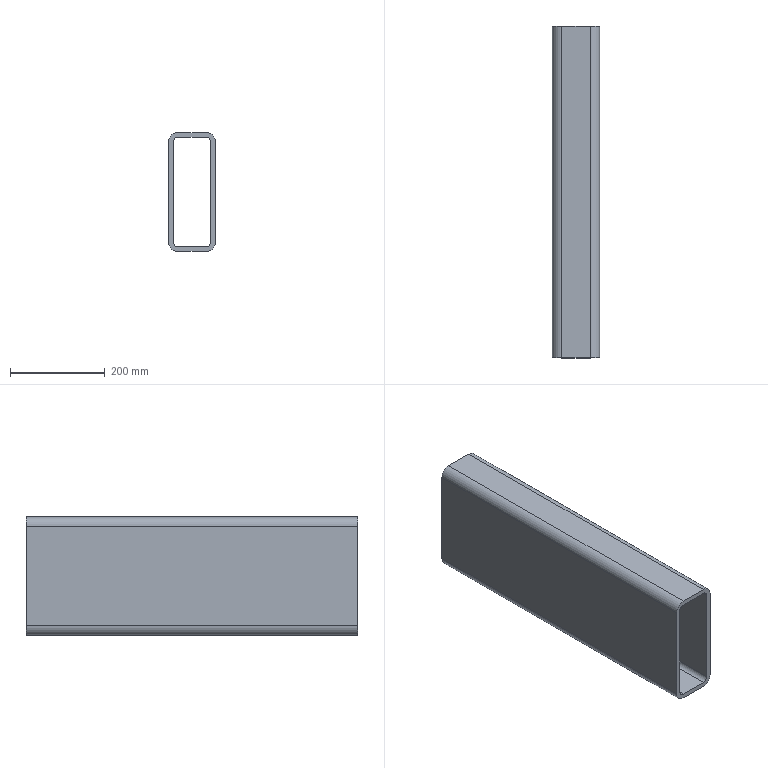Component | SolidWorks | Part10-1 | 1 solid | 18 faces | box 100 x 700 x 250 mm | volume 4439734 mm3 | plane 10 | cylinder 8 | commonest cylinder face diameters 40 x4 20 x4 | material Electroplated Steel
build123d program:
from build123d import *

# Parameters (mm, degrees)
BOSS_EXTRUDE1_DEPTH = 350


with BuildPart() as part:
    # Sketch1 → Boss-Extrude1 (new, symmetric)
    with BuildSketch(Plane.XY):
        with BuildLine():
            Line((105, -50), (-105, -50))
            ThreePointArc((-105, -50), (-119.142, -44.142), (-125, -30))
            Line((-125, -30), (-125, 30))
            ThreePointArc((-125, 30), (-119.142, 44.142), (-105, 50))
            Line((-105, 50), (105, 50))
            ThreePointArc((105, 50), (119.142, 44.142), (125, 30))
            Line((125, 30), (125, -30))
            ThreePointArc((125, -30), (119.142, -44.142), (105, -50))
        make_face()
        with BuildLine():
            Line((105, 40), (-105, 40))
            ThreePointArc((-105, 40), (-112.071, 37.071), (-115, 30))
            Line((-115, 30), (-115, -30))
            ThreePointArc((-115, -30), (-112.071, -37.071), (-105, -40))
            Line((-105, -40), (105, -40))
            ThreePointArc((105, -40), (112.071, -37.071), (115, -30))
            Line((115, -30), (115, 30))
            ThreePointArc((115, 30), (112.071, 37.071), (105, 40))
        make_face(mode=Mode.SUBTRACT)
    extrude(amount=BOSS_EXTRUDE1_DEPTH, both=True)


solid = part.part

# Placed as in the assembly
solid = solid.moved(Location((-7.456, -688.275, 505), (90, 0, 90)))
STEP:
#1=COLOUR_RGB('',0.7922,0.8196,0.9333);
#2=FILL_AREA_STYLE_COLOUR('',#1);
#3=FILL_AREA_STYLE('',(#2));
#4=SURFACE_STYLE_FILL_AREA(#3);
#5=SURFACE_SIDE_STYLE('',(#4));
#6=SURFACE_STYLE_USAGE(.BOTH.,#5);
#7=PRESENTATION_STYLE_ASSIGNMENT((#6));
#8=CARTESIAN_POINT('',(-1.475,-40.877,24.803));
#9=VERTEX_POINT('',#8);
#10=CARTESIAN_POINT('',(-2.262,-40.877,24.016));
#11=VERTEX_POINT('',#10);
#12=CARTESIAN_POINT('',(-1.475,-40.877,24.016));
#13=DIRECTION('',(0.,-1.,0.));
#14=DIRECTION('',(0.,0.,-1.));
#15=AXIS2_PLACEMENT_3D('',#12,#13,#14);
#16=CIRCLE('',#15,0.7874);
#17=EDGE_CURVE('',#9,#11,#16,.T.);
#18=ORIENTED_EDGE('',*,*,#17,.T.);
#19=CARTESIAN_POINT('',(-2.262,-40.877,15.748));
#20=VERTEX_POINT('',#19);
#21=CARTESIAN_POINT('',(-2.262,-40.877,15.748));
#22=DIRECTION('',(0.,0.,-1.));
#23=VECTOR('',#22,39.37);
#24=LINE('',#21,#23);
#25=EDGE_CURVE('',#11,#20,#24,.T.);
#26=ORIENTED_EDGE('',*,*,#25,.T.);
#27=CARTESIAN_POINT('',(-1.475,-40.877,14.961));
#28=VERTEX_POINT('',#27);
#29=CARTESIAN_POINT('',(-1.475,-40.877,15.748));
#30=DIRECTION('',(0.,-1.,0.));
#31=DIRECTION('',(0.,0.,1.));
#32=AXIS2_PLACEMENT_3D('',#29,#30,#31);
#33=CIRCLE('',#32,0.7874);
#34=EDGE_CURVE('',#20,#28,#33,.T.);
#35=ORIENTED_EDGE('',*,*,#34,.T.);
#36=CARTESIAN_POINT('',(0.8876,-40.877,14.961));
#37=VERTEX_POINT('',#36);
#38=CARTESIAN_POINT('',(-1.475,-40.877,14.961));
#39=DIRECTION('',(1.,0.,0.));
#40=VECTOR('',#39,39.37);
#41=LINE('',#38,#40);
#42=EDGE_CURVE('',#28,#37,#41,.T.);
#43=ORIENTED_EDGE('',*,*,#42,.T.);
#44=CARTESIAN_POINT('',(1.675,-40.877,15.748));
#45=VERTEX_POINT('',#44);
#46=CARTESIAN_POINT('',(0.8876,-40.877,15.748));
#47=DIRECTION('',(0.,-1.,0.));
#48=DIRECTION('',(0.,0.,-1.));
#49=AXIS2_PLACEMENT_3D('',#46,#47,#48);
#50=CIRCLE('',#49,0.7874);
#51=EDGE_CURVE('',#37,#45,#50,.T.);
#52=ORIENTED_EDGE('',*,*,#51,.T.);
#53=CARTESIAN_POINT('',(1.675,-40.877,24.016));
#54=VERTEX_POINT('',#53);
#55=CARTESIAN_POINT('',(1.675,-40.877,15.748));
#56=DIRECTION('',(-0.,-0.,1.));
#57=VECTOR('',#56,39.37);
#58=LINE('',#55,#57);
#59=EDGE_CURVE('',#45,#54,#58,.T.);
#60=ORIENTED_EDGE('',*,*,#59,.T.);
#61=CARTESIAN_POINT('',(0.8876,-40.877,24.803));
#62=VERTEX_POINT('',#61);
#63=CARTESIAN_POINT('',(0.8876,-40.877,24.016));
#64=DIRECTION('',(0.,-1.,0.));
#65=DIRECTION('',(0.,0.,-1.));
#66=AXIS2_PLACEMENT_3D('',#63,#64,#65);
#67=CIRCLE('',#66,0.7874);
#68=EDGE_CURVE('',#54,#62,#67,.T.);
#69=ORIENTED_EDGE('',*,*,#68,.T.);
#70=CARTESIAN_POINT('',(-1.475,-40.877,24.803));
#71=DIRECTION('',(-1.,-0.,0.));
#72=VECTOR('',#71,39.37);
#73=LINE('',#70,#72);
#74=EDGE_CURVE('',#62,#9,#73,.T.);
#75=ORIENTED_EDGE('',*,*,#74,.T.);
#76=EDGE_LOOP('',(#18,#26,#35,#43,#52,#60,#69,#75));
#77=FACE_OUTER_BOUND('',#76,.T.);
#78=CARTESIAN_POINT('',(1.281,-40.877,15.748));
#79=VERTEX_POINT('',#78);
#80=CARTESIAN_POINT('',(1.281,-40.877,24.016));
#81=VERTEX_POINT('',#80);
#82=CARTESIAN_POINT('',(1.281,-40.877,15.748));
#83=DIRECTION('',(0.,0.,1.));
#84=VECTOR('',#83,39.37);
#85=LINE('',#82,#84);
#86=EDGE_CURVE('',#79,#81,#85,.T.);
#87=ORIENTED_EDGE('',*,*,#86,.F.);
#88=CARTESIAN_POINT('',(0.8876,-40.877,15.354));
#89=VERTEX_POINT('',#88);
#90=CARTESIAN_POINT('',(0.8876,-40.877,15.748));
#91=DIRECTION('',(0.,-1.,0.));
#92=DIRECTION('',(0.,0.,-1.));
#93=AXIS2_PLACEMENT_3D('',#90,#91,#92);
#94=CIRCLE('',#93,0.3937);
#95=EDGE_CURVE('',#89,#79,#94,.T.);
#96=ORIENTED_EDGE('',*,*,#95,.F.);
#97=CARTESIAN_POINT('',(-1.475,-40.877,15.354));
#98=VERTEX_POINT('',#97);
#99=CARTESIAN_POINT('',(-1.475,-40.877,15.354));
#100=DIRECTION('',(1.,0.,-0.));
#101=VECTOR('',#100,39.37);
#102=LINE('',#99,#101);
#103=EDGE_CURVE('',#98,#89,#102,.T.);
#104=ORIENTED_EDGE('',*,*,#103,.F.);
#105=CARTESIAN_POINT('',(-1.868,-40.877,15.748));
#106=VERTEX_POINT('',#105);
#107=CARTESIAN_POINT('',(-1.475,-40.877,15.748));
#108=DIRECTION('',(0.,-1.,0.));
#109=DIRECTION('',(0.,0.,1.));
#110=AXIS2_PLACEMENT_3D('',#107,#108,#109);
#111=CIRCLE('',#110,0.3937);
#112=EDGE_CURVE('',#106,#98,#111,.T.);
#113=ORIENTED_EDGE('',*,*,#112,.F.);
#114=CARTESIAN_POINT('',(-1.868,-40.877,24.016));
#115=VERTEX_POINT('',#114);
#116=CARTESIAN_POINT('',(-1.868,-40.877,15.748));
#117=DIRECTION('',(0.,0.,-1.));
#118=VECTOR('',#117,39.37);
#119=LINE('',#116,#118);
#120=EDGE_CURVE('',#115,#106,#119,.T.);
#121=ORIENTED_EDGE('',*,*,#120,.F.);
#122=CARTESIAN_POINT('',(-1.475,-40.877,24.409));
#123=VERTEX_POINT('',#122);
#124=CARTESIAN_POINT('',(-1.475,-40.877,24.016));
#125=DIRECTION('',(0.,-1.,0.));
#126=DIRECTION('',(0.,0.,-1.));
#127=AXIS2_PLACEMENT_3D('',#124,#125,#126);
#128=CIRCLE('',#127,0.3937);
#129=EDGE_CURVE('',#123,#115,#128,.T.);
#130=ORIENTED_EDGE('',*,*,#129,.F.);
#131=CARTESIAN_POINT('',(0.8876,-40.877,24.409));
#132=VERTEX_POINT('',#131);
#133=CARTESIAN_POINT('',(-1.475,-40.877,24.409));
#134=DIRECTION('',(-1.,-0.,0.));
#135=VECTOR('',#134,39.37);
#136=LINE('',#133,#135);
#137=EDGE_CURVE('',#132,#123,#136,.T.);
#138=ORIENTED_EDGE('',*,*,#137,.F.);
#139=CARTESIAN_POINT('',(0.8876,-40.877,24.016));
#140=DIRECTION('',(0.,-1.,0.));
#141=DIRECTION('',(0.,0.,-1.));
#142=AXIS2_PLACEMENT_3D('',#139,#140,#141);
#143=CIRCLE('',#142,0.3937);
#144=EDGE_CURVE('',#81,#132,#143,.T.);
#145=ORIENTED_EDGE('',*,*,#144,.F.);
#146=EDGE_LOOP('',(#87,#96,#104,#113,#121,#130,#138,#145));
#147=FACE_BOUND('',#146,.T.);
#148=CARTESIAN_POINT('',(-1.475,-40.877,24.016));
#149=DIRECTION('',(0.,-1.,0.));
#150=DIRECTION('',(0.,0.,-1.));
#151=AXIS2_PLACEMENT_3D('',#148,#149,#150);
#152=PLANE('',#151);
#153=ADVANCED_FACE('',(#77,#147),#152,.T.);
#154=CARTESIAN_POINT('',(-1.475,-13.318,24.803));
#155=VERTEX_POINT('',#154);
#156=CARTESIAN_POINT('',(-2.262,-13.318,24.016));
#157=VERTEX_POINT('',#156);
#158=CARTESIAN_POINT('',(-1.475,-13.318,24.016));
#159=DIRECTION('',(0.,-1.,0.));
#160=DIRECTION('',(0.,0.,-1.));
#161=AXIS2_PLACEMENT_3D('',#158,#159,#160);
#162=CIRCLE('',#161,0.7874);
#163=EDGE_CURVE('',#155,#157,#162,.T.);
#164=ORIENTED_EDGE('',*,*,#163,.F.);
#165=CARTESIAN_POINT('',(0.8876,-13.318,24.803));
#166=VERTEX_POINT('',#165);
#167=CARTESIAN_POINT('',(-1.475,-13.318,24.803));
#168=DIRECTION('',(-1.,-0.,0.));
#169=VECTOR('',#168,39.37);
#170=LINE('',#167,#169);
#171=EDGE_CURVE('',#166,#155,#170,.T.);
#172=ORIENTED_EDGE('',*,*,#171,.F.);
#173=CARTESIAN_POINT('',(1.675,-13.318,24.016));
#174=VERTEX_POINT('',#173);
#175=CARTESIAN_POINT('',(0.8876,-13.318,24.016));
#176=DIRECTION('',(0.,-1.,0.));
#177=DIRECTION('',(0.,0.,-1.));
#178=AXIS2_PLACEMENT_3D('',#175,#176,#177);
#179=CIRCLE('',#178,0.7874);
#180=EDGE_CURVE('',#174,#166,#179,.T.);
#181=ORIENTED_EDGE('',*,*,#180,.F.);
#182=CARTESIAN_POINT('',(1.675,-13.318,15.748));
#183=VERTEX_POINT('',#182);
#184=CARTESIAN_POINT('',(1.675,-13.318,15.748));
#185=DIRECTION('',(-0.,-0.,1.));
#186=VECTOR('',#185,39.37);
#187=LINE('',#184,#186);
#188=EDGE_CURVE('',#183,#174,#187,.T.);
#189=ORIENTED_EDGE('',*,*,#188,.F.);
#190=CARTESIAN_POINT('',(0.8876,-13.318,14.961));
#191=VERTEX_POINT('',#190);
#192=CARTESIAN_POINT('',(0.8876,-13.318,15.748));
#193=DIRECTION('',(0.,-1.,0.));
#194=DIRECTION('',(0.,0.,-1.));
#195=AXIS2_PLACEMENT_3D('',#192,#193,#194);
#196=CIRCLE('',#195,0.7874);
#197=EDGE_CURVE('',#191,#183,#196,.T.);
#198=ORIENTED_EDGE('',*,*,#197,.F.);
#199=CARTESIAN_POINT('',(-1.475,-13.318,14.961));
#200=VERTEX_POINT('',#199);
#201=CARTESIAN_POINT('',(-1.475,-13.318,14.961));
#202=DIRECTION('',(1.,0.,0.));
#203=VECTOR('',#202,39.37);
#204=LINE('',#201,#203);
#205=EDGE_CURVE('',#200,#191,#204,.T.);
#206=ORIENTED_EDGE('',*,*,#205,.F.);
#207=CARTESIAN_POINT('',(-2.262,-13.318,15.748));
#208=VERTEX_POINT('',#207);
#209=CARTESIAN_POINT('',(-1.475,-13.318,15.748));
#210=DIRECTION('',(0.,-1.,0.));
#211=DIRECTION('',(0.,0.,1.));
#212=AXIS2_PLACEMENT_3D('',#209,#210,#211);
#213=CIRCLE('',#212,0.7874);
#214=EDGE_CURVE('',#208,#200,#213,.T.);
#215=ORIENTED_EDGE('',*,*,#214,.F.);
#216=CARTESIAN_POINT('',(-2.262,-13.318,15.748));
#217=DIRECTION('',(0.,0.,-1.));
#218=VECTOR('',#217,39.37);
#219=LINE('',#216,#218);
#220=EDGE_CURVE('',#157,#208,#219,.T.);
#221=ORIENTED_EDGE('',*,*,#220,.F.);
#222=EDGE_LOOP('',(#164,#172,#181,#189,#198,#206,#215,#221));
#223=FACE_OUTER_BOUND('',#222,.T.);
#224=CARTESIAN_POINT('',(0.8876,-13.318,15.354));
#225=VERTEX_POINT('',#224);
#226=CARTESIAN_POINT('',(1.281,-13.318,15.748));
#227=VERTEX_POINT('',#226);
#228=CARTESIAN_POINT('',(0.8876,-13.318,15.748));
#229=DIRECTION('',(0.,-1.,0.));
#230=DIRECTION('',(0.,0.,-1.));
#231=AXIS2_PLACEMENT_3D('',#228,#229,#230);
#232=CIRCLE('',#231,0.3937);
#233=EDGE_CURVE('',#225,#227,#232,.T.);
#234=ORIENTED_EDGE('',*,*,#233,.T.);
#235=CARTESIAN_POINT('',(1.281,-13.318,24.016));
#236=VERTEX_POINT('',#235);
#237=CARTESIAN_POINT('',(1.281,-13.318,15.748));
#238=DIRECTION('',(0.,0.,1.));
#239=VECTOR('',#238,39.37);
#240=LINE('',#237,#239);
#241=EDGE_CURVE('',#227,#236,#240,.T.);
#242=ORIENTED_EDGE('',*,*,#241,.T.);
#243=CARTESIAN_POINT('',(0.8876,-13.318,24.409));
#244=VERTEX_POINT('',#243);
#245=CARTESIAN_POINT('',(0.8876,-13.318,24.016));
#246=DIRECTION('',(0.,-1.,0.));
#247=DIRECTION('',(0.,0.,-1.));
#248=AXIS2_PLACEMENT_3D('',#245,#246,#247);
#249=CIRCLE('',#248,0.3937);
#250=EDGE_CURVE('',#236,#244,#249,.T.);
#251=ORIENTED_EDGE('',*,*,#250,.T.);
#252=CARTESIAN_POINT('',(-1.475,-13.318,24.409));
#253=VERTEX_POINT('',#252);
#254=CARTESIAN_POINT('',(-1.475,-13.318,24.409));
#255=DIRECTION('',(-1.,-0.,0.));
#256=VECTOR('',#255,39.37);
#257=LINE('',#254,#256);
#258=EDGE_CURVE('',#244,#253,#257,.T.);
#259=ORIENTED_EDGE('',*,*,#258,.T.);
#260=CARTESIAN_POINT('',(-1.868,-13.318,24.016));
#261=VERTEX_POINT('',#260);
#262=CARTESIAN_POINT('',(-1.475,-13.318,24.016));
#263=DIRECTION('',(0.,-1.,0.));
#264=DIRECTION('',(0.,0.,-1.));
#265=AXIS2_PLACEMENT_3D('',#262,#263,#264);
#266=CIRCLE('',#265,0.3937);
#267=EDGE_CURVE('',#253,#261,#266,.T.);
#268=ORIENTED_EDGE('',*,*,#267,.T.);
#269=CARTESIAN_POINT('',(-1.868,-13.318,15.748));
#270=VERTEX_POINT('',#269);
#271=CARTESIAN_POINT('',(-1.868,-13.318,15.748));
#272=DIRECTION('',(0.,0.,-1.));
#273=VECTOR('',#272,39.37);
#274=LINE('',#271,#273);
#275=EDGE_CURVE('',#261,#270,#274,.T.);
#276=ORIENTED_EDGE('',*,*,#275,.T.);
#277=CARTESIAN_POINT('',(-1.475,-13.318,15.354));
#278=VERTEX_POINT('',#277);
#279=CARTESIAN_POINT('',(-1.475,-13.318,15.748));
#280=DIRECTION('',(0.,-1.,0.));
#281=DIRECTION('',(0.,0.,1.));
#282=AXIS2_PLACEMENT_3D('',#279,#280,#281);
#283=CIRCLE('',#282,0.3937);
#284=EDGE_CURVE('',#270,#278,#283,.T.);
#285=ORIENTED_EDGE('',*,*,#284,.T.);
#286=CARTESIAN_POINT('',(-1.475,-13.318,15.354));
#287=DIRECTION('',(1.,0.,-0.));
#288=VECTOR('',#287,39.37);
#289=LINE('',#286,#288);
#290=EDGE_CURVE('',#278,#225,#289,.T.);
#291=ORIENTED_EDGE('',*,*,#290,.T.);
#292=EDGE_LOOP('',(#234,#242,#251,#259,#268,#276,#285,#291));
#293=FACE_BOUND('',#292,.T.);
#294=CARTESIAN_POINT('',(-1.475,-13.318,24.016));
#295=DIRECTION('',(0.,-1.,0.));
#296=DIRECTION('',(0.,0.,-1.));
#297=AXIS2_PLACEMENT_3D('',#294,#295,#296);
#298=PLANE('',#297);
#299=ADVANCED_FACE('',(#223,#293),#298,.F.);
#300=ORIENTED_EDGE('',*,*,#163,.T.);
#301=CARTESIAN_POINT('',(-2.262,-40.877,24.016));
#302=DIRECTION('',(-0.,1.,0.));
#303=VECTOR('',#302,39.37);
#304=LINE('',#301,#303);
#305=EDGE_CURVE('',#11,#157,#304,.T.);
#306=ORIENTED_EDGE('',*,*,#305,.F.);
#307=ORIENTED_EDGE('',*,*,#17,.F.);
#308=CARTESIAN_POINT('',(-1.475,-40.877,24.803));
#309=DIRECTION('',(-0.,1.,0.));
#310=VECTOR('',#309,39.37);
#311=LINE('',#308,#310);
#312=EDGE_CURVE('',#9,#155,#311,.T.);
#313=ORIENTED_EDGE('',*,*,#312,.T.);
#314=EDGE_LOOP('',(#300,#306,#307,#313));
#315=FACE_OUTER_BOUND('',#314,.T.);
#316=CARTESIAN_POINT('',(-1.475,-40.877,24.016));
#317=DIRECTION('',(-0.,1.,0.));
#318=DIRECTION('',(0.,0.,1.));
#319=AXIS2_PLACEMENT_3D('',#316,#317,#318);
#320=CYLINDRICAL_SURFACE('',#319,0.7874);
#321=ADVANCED_FACE('',(#315),#320,.T.);
#322=ORIENTED_EDGE('',*,*,#220,.T.);
#323=CARTESIAN_POINT('',(-2.262,-40.877,15.748));
#324=DIRECTION('',(-0.,1.,0.));
#325=VECTOR('',#324,39.37);
#326=LINE('',#323,#325);
#327=EDGE_CURVE('',#20,#208,#326,.T.);
#328=ORIENTED_EDGE('',*,*,#327,.F.);
#329=ORIENTED_EDGE('',*,*,#25,.F.);
#330=ORIENTED_EDGE('',*,*,#305,.T.);
#331=EDGE_LOOP('',(#322,#328,#329,#330));
#332=FACE_OUTER_BOUND('',#331,.T.);
#333=CARTESIAN_POINT('',(-2.262,-40.877,15.748));
#334=DIRECTION('',(1.,0.,0.));
#335=DIRECTION('',(-0.,-0.,1.));
#336=AXIS2_PLACEMENT_3D('',#333,#334,#335);
#337=PLANE('',#336);
#338=ADVANCED_FACE('',(#332),#337,.F.);
#339=ORIENTED_EDGE('',*,*,#214,.T.);
#340=CARTESIAN_POINT('',(-1.475,-40.877,14.961));
#341=DIRECTION('',(-0.,1.,0.));
#342=VECTOR('',#341,39.37);
#343=LINE('',#340,#342);
#344=EDGE_CURVE('',#28,#200,#343,.T.);
#345=ORIENTED_EDGE('',*,*,#344,.F.);
#346=ORIENTED_EDGE('',*,*,#34,.F.);
#347=ORIENTED_EDGE('',*,*,#327,.T.);
#348=EDGE_LOOP('',(#339,#345,#346,#347));
#349=FACE_OUTER_BOUND('',#348,.T.);
#350=CARTESIAN_POINT('',(-1.475,-40.877,15.748));
#351=DIRECTION('',(-0.,1.,0.));
#352=DIRECTION('',(0.,0.,1.));
#353=AXIS2_PLACEMENT_3D('',#350,#351,#352);
#354=CYLINDRICAL_SURFACE('',#353,0.7874);
#355=ADVANCED_FACE('',(#349),#354,.T.);
#356=ORIENTED_EDGE('',*,*,#205,.T.);
#357=CARTESIAN_POINT('',(0.8876,-40.877,14.961));
#358=DIRECTION('',(-0.,1.,0.));
#359=VECTOR('',#358,39.37);
#360=LINE('',#357,#359);
#361=EDGE_CURVE('',#37,#191,#360,.T.);
#362=ORIENTED_EDGE('',*,*,#361,.F.);
#363=ORIENTED_EDGE('',*,*,#42,.F.);
#364=ORIENTED_EDGE('',*,*,#344,.T.);
#365=EDGE_LOOP('',(#356,#362,#363,#364));
#366=FACE_OUTER_BOUND('',#365,.T.);
#367=CARTESIAN_POINT('',(-1.475,-40.877,14.961));
#368=DIRECTION('',(0.,0.,1.));
#369=DIRECTION('',(0.,-1.,0.));
#370=AXIS2_PLACEMENT_3D('',#367,#368,#369);
#371=PLANE('',#370);
#372=ADVANCED_FACE('',(#366),#371,.F.);
#373=ORIENTED_EDGE('',*,*,#197,.T.);
#374=CARTESIAN_POINT('',(1.675,-40.877,15.748));
#375=DIRECTION('',(-0.,1.,0.));
#376=VECTOR('',#375,39.37);
#377=LINE('',#374,#376);
#378=EDGE_CURVE('',#45,#183,#377,.T.);
#379=ORIENTED_EDGE('',*,*,#378,.F.);
#380=ORIENTED_EDGE('',*,*,#51,.F.);
#381=ORIENTED_EDGE('',*,*,#361,.T.);
#382=EDGE_LOOP('',(#373,#379,#380,#381));
#383=FACE_OUTER_BOUND('',#382,.T.);
#384=CARTESIAN_POINT('',(0.8876,-40.877,15.748));
#385=DIRECTION('',(-0.,1.,0.));
#386=DIRECTION('',(0.,0.,1.));
#387=AXIS2_PLACEMENT_3D('',#384,#385,#386);
#388=CYLINDRICAL_SURFACE('',#387,0.7874);
#389=ADVANCED_FACE('',(#383),#388,.T.);
#390=ORIENTED_EDGE('',*,*,#188,.T.);
#391=CARTESIAN_POINT('',(1.675,-40.877,24.016));
#392=DIRECTION('',(-0.,1.,0.));
#393=VECTOR('',#392,39.37);
#394=LINE('',#391,#393);
#395=EDGE_CURVE('',#54,#174,#394,.T.);
#396=ORIENTED_EDGE('',*,*,#395,.F.);
#397=ORIENTED_EDGE('',*,*,#59,.F.);
#398=ORIENTED_EDGE('',*,*,#378,.T.);
#399=EDGE_LOOP('',(#390,#396,#397,#398));
#400=FACE_OUTER_BOUND('',#399,.T.);
#401=CARTESIAN_POINT('',(1.675,-40.877,15.748));
#402=DIRECTION('',(-1.,-0.,-0.));
#403=DIRECTION('',(0.,0.,-1.));
#404=AXIS2_PLACEMENT_3D('',#401,#402,#403);
#405=PLANE('',#404);
#406=ADVANCED_FACE('',(#400),#405,.F.);
#407=ORIENTED_EDGE('',*,*,#180,.T.);
#408=CARTESIAN_POINT('',(0.8876,-40.877,24.803));
#409=DIRECTION('',(-0.,1.,0.));
#410=VECTOR('',#409,39.37);
#411=LINE('',#408,#410);
#412=EDGE_CURVE('',#62,#166,#411,.T.);
#413=ORIENTED_EDGE('',*,*,#412,.F.);
#414=ORIENTED_EDGE('',*,*,#68,.F.);
#415=ORIENTED_EDGE('',*,*,#395,.T.);
#416=EDGE_LOOP('',(#407,#413,#414,#415));
#417=FACE_OUTER_BOUND('',#416,.T.);
#418=CARTESIAN_POINT('',(0.8876,-40.877,24.016));
#419=DIRECTION('',(-0.,1.,0.));
#420=DIRECTION('',(0.,0.,1.));
#421=AXIS2_PLACEMENT_3D('',#418,#419,#420);
#422=CYLINDRICAL_SURFACE('',#421,0.7874);
#423=ADVANCED_FACE('',(#417),#422,.T.);
#424=ORIENTED_EDGE('',*,*,#171,.T.);
#425=ORIENTED_EDGE('',*,*,#312,.F.);
#426=ORIENTED_EDGE('',*,*,#74,.F.);
#427=ORIENTED_EDGE('',*,*,#412,.T.);
#428=EDGE_LOOP('',(#424,#425,#426,#427));
#429=FACE_OUTER_BOUND('',#428,.T.);
#430=CARTESIAN_POINT('',(-1.475,-40.877,24.803));
#431=DIRECTION('',(0.,0.,-1.));
#432=DIRECTION('',(-0.,1.,0.));
#433=AXIS2_PLACEMENT_3D('',#430,#431,#432);
#434=PLANE('',#433);
#435=ADVANCED_FACE('',(#429),#434,.F.);
#436=ORIENTED_EDGE('',*,*,#233,.F.);
#437=CARTESIAN_POINT('',(0.8876,-40.877,15.354));
#438=DIRECTION('',(-0.,1.,0.));
#439=VECTOR('',#438,39.37);
#440=LINE('',#437,#439);
#441=EDGE_CURVE('',#89,#225,#440,.T.);
#442=ORIENTED_EDGE('',*,*,#441,.F.);
#443=ORIENTED_EDGE('',*,*,#95,.T.);
#444=CARTESIAN_POINT('',(1.281,-40.877,15.748));
#445=DIRECTION('',(-0.,1.,0.));
#446=VECTOR('',#445,39.37);
#447=LINE('',#444,#446);
#448=EDGE_CURVE('',#79,#227,#447,.T.);
#449=ORIENTED_EDGE('',*,*,#448,.T.);
#450=EDGE_LOOP('',(#436,#442,#443,#449));
#451=FACE_OUTER_BOUND('',#450,.T.);
#452=CARTESIAN_POINT('',(0.8876,-40.877,15.748));
#453=DIRECTION('',(-0.,1.,0.));
#454=DIRECTION('',(0.,0.,1.));
#455=AXIS2_PLACEMENT_3D('',#452,#453,#454);
#456=CYLINDRICAL_SURFACE('',#455,0.3937);
#457=ADVANCED_FACE('',(#451),#456,.F.);
#458=ORIENTED_EDGE('',*,*,#241,.F.);
#459=ORIENTED_EDGE('',*,*,#448,.F.);
#460=ORIENTED_EDGE('',*,*,#86,.T.);
#461=CARTESIAN_POINT('',(1.281,-40.877,24.016));
#462=DIRECTION('',(-0.,1.,0.));
#463=VECTOR('',#462,39.37);
#464=LINE('',#461,#463);
#465=EDGE_CURVE('',#81,#236,#464,.T.);
#466=ORIENTED_EDGE('',*,*,#465,.T.);
#467=EDGE_LOOP('',(#458,#459,#460,#466));
#468=FACE_OUTER_BOUND('',#467,.T.);
#469=CARTESIAN_POINT('',(1.281,-40.877,15.748));
#470=DIRECTION('',(-1.,-0.,0.));
#471=DIRECTION('',(-0.,1.,0.));
#472=AXIS2_PLACEMENT_3D('',#469,#470,#471);
#473=PLANE('',#472);
#474=ADVANCED_FACE('',(#468),#473,.T.);
#475=ORIENTED_EDGE('',*,*,#250,.F.);
#476=ORIENTED_EDGE('',*,*,#465,.F.);
#477=ORIENTED_EDGE('',*,*,#144,.T.);
#478=CARTESIAN_POINT('',(0.8876,-40.877,24.409));
#479=DIRECTION('',(-0.,1.,0.));
#480=VECTOR('',#479,39.37);
#481=LINE('',#478,#480);
#482=EDGE_CURVE('',#132,#244,#481,.T.);
#483=ORIENTED_EDGE('',*,*,#482,.T.);
#484=EDGE_LOOP('',(#475,#476,#477,#483));
#485=FACE_OUTER_BOUND('',#484,.T.);
#486=CARTESIAN_POINT('',(0.8876,-40.877,24.016));
#487=DIRECTION('',(-0.,1.,0.));
#488=DIRECTION('',(0.,0.,1.));
#489=AXIS2_PLACEMENT_3D('',#486,#487,#488);
#490=CYLINDRICAL_SURFACE('',#489,0.3937);
#491=ADVANCED_FACE('',(#485),#490,.F.);
#492=ORIENTED_EDGE('',*,*,#258,.F.);
#493=ORIENTED_EDGE('',*,*,#482,.F.);
#494=ORIENTED_EDGE('',*,*,#137,.T.);
#495=CARTESIAN_POINT('',(-1.475,-40.877,24.409));
#496=DIRECTION('',(-0.,1.,0.));
#497=VECTOR('',#496,39.37);
#498=LINE('',#495,#497);
#499=EDGE_CURVE('',#123,#253,#498,.T.);
#500=ORIENTED_EDGE('',*,*,#499,.T.);
#501=EDGE_LOOP('',(#492,#493,#494,#500));
#502=FACE_OUTER_BOUND('',#501,.T.);
#503=CARTESIAN_POINT('',(-1.475,-40.877,24.409));
#504=DIRECTION('',(-0.,-0.,-1.));
#505=DIRECTION('',(1.,0.,-0.));
#506=AXIS2_PLACEMENT_3D('',#503,#504,#505);
#507=PLANE('',#506);
#508=ADVANCED_FACE('',(#502),#507,.T.);
#509=ORIENTED_EDGE('',*,*,#267,.F.);
#510=ORIENTED_EDGE('',*,*,#499,.F.);
#511=ORIENTED_EDGE('',*,*,#129,.T.);
#512=CARTESIAN_POINT('',(-1.868,-40.877,24.016));
#513=DIRECTION('',(-0.,1.,0.));
#514=VECTOR('',#513,39.37);
#515=LINE('',#512,#514);
#516=EDGE_CURVE('',#115,#261,#515,.T.);
#517=ORIENTED_EDGE('',*,*,#516,.T.);
#518=EDGE_LOOP('',(#509,#510,#511,#517));
#519=FACE_OUTER_BOUND('',#518,.T.);
#520=CARTESIAN_POINT('',(-1.475,-40.877,24.016));
#521=DIRECTION('',(-0.,1.,0.));
#522=DIRECTION('',(0.,0.,1.));
#523=AXIS2_PLACEMENT_3D('',#520,#521,#522);
#524=CYLINDRICAL_SURFACE('',#523,0.3937);
#525=ADVANCED_FACE('',(#519),#524,.F.);
#526=ORIENTED_EDGE('',*,*,#275,.F.);
#527=ORIENTED_EDGE('',*,*,#516,.F.);
#528=ORIENTED_EDGE('',*,*,#120,.T.);
#529=CARTESIAN_POINT('',(-1.868,-40.877,15.748));
#530=DIRECTION('',(-0.,1.,0.));
#531=VECTOR('',#530,39.37);
#532=LINE('',#529,#531);
#533=EDGE_CURVE('',#106,#270,#532,.T.);
#534=ORIENTED_EDGE('',*,*,#533,.T.);
#535=EDGE_LOOP('',(#526,#527,#528,#534));
#536=FACE_OUTER_BOUND('',#535,.T.);
#537=CARTESIAN_POINT('',(-1.868,-40.877,15.748));
#538=DIRECTION('',(1.,0.,0.));
#539=DIRECTION('',(-0.,-0.,1.));
#540=AXIS2_PLACEMENT_3D('',#537,#538,#539);
#541=PLANE('',#540);
#542=ADVANCED_FACE('',(#536),#541,.T.);
#543=ORIENTED_EDGE('',*,*,#284,.F.);
#544=ORIENTED_EDGE('',*,*,#533,.F.);
#545=ORIENTED_EDGE('',*,*,#112,.T.);
#546=CARTESIAN_POINT('',(-1.475,-40.877,15.354));
#547=DIRECTION('',(-0.,1.,0.));
#548=VECTOR('',#547,39.37);
#549=LINE('',#546,#548);
#550=EDGE_CURVE('',#98,#278,#549,.T.);
#551=ORIENTED_EDGE('',*,*,#550,.T.);
#552=EDGE_LOOP('',(#543,#544,#545,#551));
#553=FACE_OUTER_BOUND('',#552,.T.);
#554=CARTESIAN_POINT('',(-1.475,-40.877,15.748));
#555=DIRECTION('',(-0.,1.,0.));
#556=DIRECTION('',(0.,0.,1.));
#557=AXIS2_PLACEMENT_3D('',#554,#555,#556);
#558=CYLINDRICAL_SURFACE('',#557,0.3937);
#559=ADVANCED_FACE('',(#553),#558,.F.);
#560=ORIENTED_EDGE('',*,*,#290,.F.);
#561=ORIENTED_EDGE('',*,*,#550,.F.);
#562=ORIENTED_EDGE('',*,*,#103,.T.);
#563=ORIENTED_EDGE('',*,*,#441,.T.);
#564=EDGE_LOOP('',(#560,#561,#562,#563));
#565=FACE_OUTER_BOUND('',#564,.T.);
#566=CARTESIAN_POINT('',(-1.475,-40.877,15.354));
#567=DIRECTION('',(0.,0.,1.));
#568=DIRECTION('',(-1.,-0.,0.));
#569=AXIS2_PLACEMENT_3D('',#566,#567,#568);
#570=PLANE('',#569);
#571=ADVANCED_FACE('',(#565),#570,.T.);
#572=CLOSED_SHELL('',(#153,#299,#321,#338,#355,#372,#389,#406,#423,#435,#457,#474,#491,#508,#525,#542,#559,#571));
#573=MANIFOLD_SOLID_BREP('',#572);
#574=STYLED_ITEM('',(#7),#573);
#575=PRESENTATION_LAYER_ASSIGNMENT('','',(#574));
#576=CARTESIAN_POINT('',(0.,0.,0.));
#577=DIRECTION('',(0.,0.,1.));
#578=DIRECTION('',(1.,0.,0.));
#579=AXIS2_PLACEMENT_3D('',#576,#577,#578);
#580=(LENGTH_UNIT()NAMED_UNIT(*)SI_UNIT($,.METRE.));
#581=LENGTH_MEASURE_WITH_UNIT(LENGTH_MEASURE(0.0254),#580);
#582=DIMENSIONAL_EXPONENTS(1.,0.,0.,0.,0.,0.,0.);
#583=(CONVERSION_BASED_UNIT('',#581)LENGTH_UNIT()NAMED_UNIT(#582));
#584=UNCERTAINTY_MEASURE_WITH_UNIT(LENGTH_MEASURE(0.00001),#583,'','');
#585=(NAMED_UNIT(*)PLANE_ANGLE_UNIT()SI_UNIT($,.RADIAN.));
#586=(NAMED_UNIT(*)SI_UNIT($,.STERADIAN.)SOLID_ANGLE_UNIT());
#587=(GEOMETRIC_REPRESENTATION_CONTEXT(3)GLOBAL_UNCERTAINTY_ASSIGNED_CONTEXT((#584))GLOBAL_UNIT_ASSIGNED_CONTEXT((#583,#585,#586))REPRESENTATION_CONTEXT('',''));
#588=ADVANCED_BREP_SHAPE_REPRESENTATION('',(#573,#579),#587);
#589=(LENGTH_UNIT()NAMED_UNIT(*)SI_UNIT($,.METRE.));
#590=LENGTH_MEASURE_WITH_UNIT(LENGTH_MEASURE(0.0254),#589);
#591=DIMENSIONAL_EXPONENTS(1.,0.,0.,0.,0.,0.,0.);
#592=(CONVERSION_BASED_UNIT('',#590)LENGTH_UNIT()NAMED_UNIT(#591));
#593=UNCERTAINTY_MEASURE_WITH_UNIT(LENGTH_MEASURE(0.00001),#592,'','');
#594=(NAMED_UNIT(*)PLANE_ANGLE_UNIT()SI_UNIT($,.RADIAN.));
#595=(NAMED_UNIT(*)SI_UNIT($,.STERADIAN.)SOLID_ANGLE_UNIT());
#596=(GEOMETRIC_REPRESENTATION_CONTEXT(3)GLOBAL_UNCERTAINTY_ASSIGNED_CONTEXT((#593))GLOBAL_UNIT_ASSIGNED_CONTEXT((#592,#594,#595))REPRESENTATION_CONTEXT('',''));
#597=MECHANICAL_DESIGN_GEOMETRIC_PRESENTATION_REPRESENTATION('',(#574),#596);